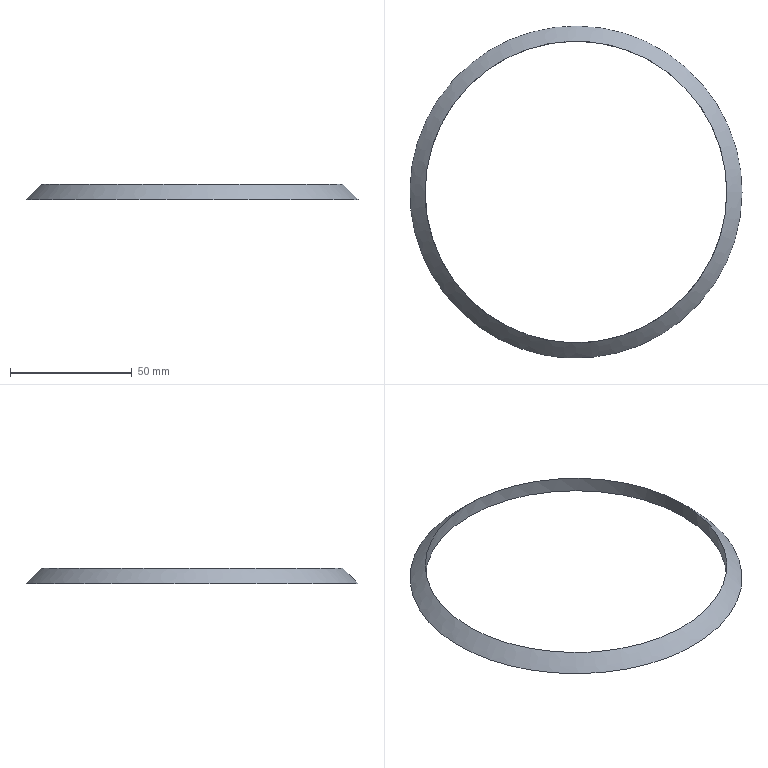Component | NX | CH3404_8_2 | 1 solid | 3 faces | volume 7866 mm3 | spline 1 | plane 1 | cylinder 1 | commonest cylinder face diameters 124 x1